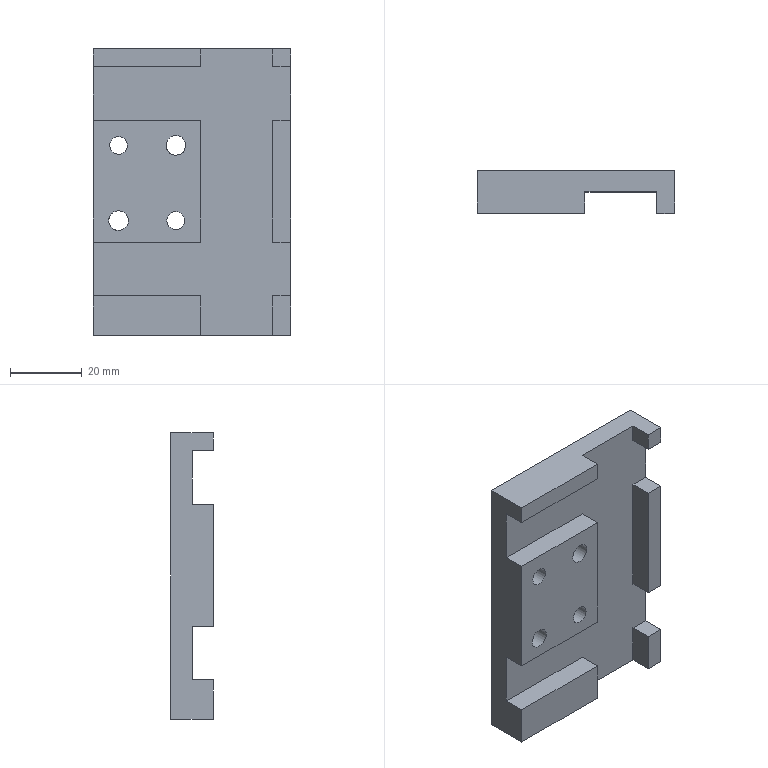Component | NX | GROOVE_GUIDE_BLOCK | 1 solid | 34 faces | volume 35234 mm3 | plane 28 | cylinder 6 | commonest cylinder face diameters 5.5 x2 10 x2 5 x2